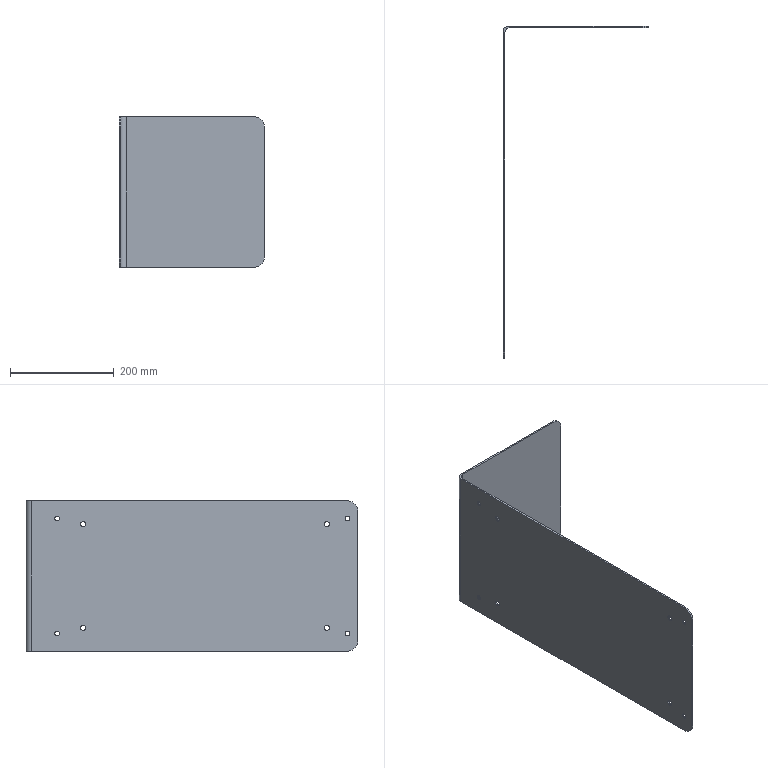Component | SolidWorks | 315InverterBracket()-1 | 1 solid | 30 faces | box 280 x 640 x 290 mm | volume 795054 mm3 | cylinder 22 | plane 8 | commonest cylinder face diameters 10 x8 9 x8 40 x4 20 x2 | material Plain Carbon Steel
STEP:
#1=COLOUR_RGB('',0.7922,0.8196,0.9333);
#2=FILL_AREA_STYLE_COLOUR('',#1);
#3=FILL_AREA_STYLE('',(#2));
#4=SURFACE_STYLE_FILL_AREA(#3);
#5=SURFACE_SIDE_STYLE('',(#4));
#6=SURFACE_STYLE_USAGE(.BOTH.,#5);
#7=PRESENTATION_STYLE_ASSIGNMENT((#6));
#8=CARTESIAN_POINT('',(26.575,78.937,-63.15));
#9=VERTEX_POINT('',#8);
#10=CARTESIAN_POINT('',(26.575,79.331,-63.15));
#11=VERTEX_POINT('',#10);
#12=CARTESIAN_POINT('',(26.575,79.134,-63.15));
#13=DIRECTION('',(-1.,0.,0.));
#14=DIRECTION('',(0.,-1.,0.));
#15=AXIS2_PLACEMENT_3D('',#12,#13,#14);
#16=CIRCLE('',#15,0.1969);
#17=EDGE_CURVE('',#9,#11,#16,.T.);
#18=ORIENTED_EDGE('',*,*,#17,.T.);
#19=CARTESIAN_POINT('',(26.693,79.331,-63.15));
#20=VERTEX_POINT('',#19);
#21=CARTESIAN_POINT('',(26.693,79.331,-63.15));
#22=DIRECTION('',(1.,-0.,-0.));
#23=VECTOR('',#22,39.37);
#24=LINE('',#21,#23);
#25=EDGE_CURVE('',#11,#20,#24,.T.);
#26=ORIENTED_EDGE('',*,*,#25,.T.);
#27=CARTESIAN_POINT('',(26.693,78.937,-63.15));
#28=VERTEX_POINT('',#27);
#29=CARTESIAN_POINT('',(26.693,79.134,-63.15));
#30=DIRECTION('',(-1.,0.,0.));
#31=DIRECTION('',(0.,-1.,0.));
#32=AXIS2_PLACEMENT_3D('',#29,#30,#31);
#33=CIRCLE('',#32,0.1969);
#34=EDGE_CURVE('',#28,#20,#33,.T.);
#35=ORIENTED_EDGE('',*,*,#34,.F.);
#36=CARTESIAN_POINT('',(26.693,78.937,-63.15));
#37=DIRECTION('',(1.,-0.,-0.));
#38=VECTOR('',#37,39.37);
#39=LINE('',#36,#38);
#40=EDGE_CURVE('',#9,#28,#39,.T.);
#41=ORIENTED_EDGE('',*,*,#40,.F.);
#42=EDGE_LOOP('',(#18,#26,#35,#41));
#43=FACE_OUTER_BOUND('',#42,.T.);
#44=CARTESIAN_POINT('',(26.693,79.134,-63.15));
#45=DIRECTION('',(1.,-0.,-0.));
#46=DIRECTION('',(0.,-1.,0.));
#47=AXIS2_PLACEMENT_3D('',#44,#45,#46);
#48=CYLINDRICAL_SURFACE('',#47,0.1969);
#49=ADVANCED_FACE('',(#43),#48,.F.);
#50=CARTESIAN_POINT('',(26.575,78.937,-71.024));
#51=VERTEX_POINT('',#50);
#52=CARTESIAN_POINT('',(26.575,79.331,-71.024));
#53=VERTEX_POINT('',#52);
#54=CARTESIAN_POINT('',(26.575,79.134,-71.024));
#55=DIRECTION('',(-1.,0.,0.));
#56=DIRECTION('',(0.,-1.,0.));
#57=AXIS2_PLACEMENT_3D('',#54,#55,#56);
#58=CIRCLE('',#57,0.1969);
#59=EDGE_CURVE('',#51,#53,#58,.T.);
#60=ORIENTED_EDGE('',*,*,#59,.T.);
#61=CARTESIAN_POINT('',(26.693,79.331,-71.024));
#62=VERTEX_POINT('',#61);
#63=CARTESIAN_POINT('',(26.693,79.331,-71.024));
#64=DIRECTION('',(1.,-0.,-0.));
#65=VECTOR('',#64,39.37);
#66=LINE('',#63,#65);
#67=EDGE_CURVE('',#53,#62,#66,.T.);
#68=ORIENTED_EDGE('',*,*,#67,.T.);
#69=CARTESIAN_POINT('',(26.693,78.937,-71.024));
#70=VERTEX_POINT('',#69);
#71=CARTESIAN_POINT('',(26.693,79.134,-71.024));
#72=DIRECTION('',(-1.,0.,0.));
#73=DIRECTION('',(0.,-1.,0.));
#74=AXIS2_PLACEMENT_3D('',#71,#72,#73);
#75=CIRCLE('',#74,0.1969);
#76=EDGE_CURVE('',#70,#62,#75,.T.);
#77=ORIENTED_EDGE('',*,*,#76,.F.);
#78=CARTESIAN_POINT('',(26.693,78.937,-71.024));
#79=DIRECTION('',(1.,-0.,-0.));
#80=VECTOR('',#79,39.37);
#81=LINE('',#78,#80);
#82=EDGE_CURVE('',#51,#70,#81,.T.);
#83=ORIENTED_EDGE('',*,*,#82,.F.);
#84=EDGE_LOOP('',(#60,#68,#77,#83));
#85=FACE_OUTER_BOUND('',#84,.T.);
#86=CARTESIAN_POINT('',(26.693,79.134,-71.024));
#87=DIRECTION('',(1.,-0.,-0.));
#88=DIRECTION('',(0.,-1.,0.));
#89=AXIS2_PLACEMENT_3D('',#86,#87,#88);
#90=CYLINDRICAL_SURFACE('',#89,0.1969);
#91=ADVANCED_FACE('',(#85),#90,.F.);
#92=CARTESIAN_POINT('',(26.575,97.441,-71.024));
#93=VERTEX_POINT('',#92);
#94=CARTESIAN_POINT('',(26.575,97.835,-71.024));
#95=VERTEX_POINT('',#94);
#96=CARTESIAN_POINT('',(26.575,97.638,-71.024));
#97=DIRECTION('',(-1.,0.,0.));
#98=DIRECTION('',(0.,-1.,0.));
#99=AXIS2_PLACEMENT_3D('',#96,#97,#98);
#100=CIRCLE('',#99,0.1969);
#101=EDGE_CURVE('',#93,#95,#100,.T.);
#102=ORIENTED_EDGE('',*,*,#101,.T.);
#103=CARTESIAN_POINT('',(26.693,97.835,-71.024));
#104=VERTEX_POINT('',#103);
#105=CARTESIAN_POINT('',(26.693,97.835,-71.024));
#106=DIRECTION('',(1.,-0.,-0.));
#107=VECTOR('',#106,39.37);
#108=LINE('',#105,#107);
#109=EDGE_CURVE('',#95,#104,#108,.T.);
#110=ORIENTED_EDGE('',*,*,#109,.T.);
#111=CARTESIAN_POINT('',(26.693,97.441,-71.024));
#112=VERTEX_POINT('',#111);
#113=CARTESIAN_POINT('',(26.693,97.638,-71.024));
#114=DIRECTION('',(-1.,0.,0.));
#115=DIRECTION('',(0.,-1.,0.));
#116=AXIS2_PLACEMENT_3D('',#113,#114,#115);
#117=CIRCLE('',#116,0.1969);
#118=EDGE_CURVE('',#112,#104,#117,.T.);
#119=ORIENTED_EDGE('',*,*,#118,.F.);
#120=CARTESIAN_POINT('',(26.693,97.441,-71.024));
#121=DIRECTION('',(1.,-0.,-0.));
#122=VECTOR('',#121,39.37);
#123=LINE('',#120,#122);
#124=EDGE_CURVE('',#93,#112,#123,.T.);
#125=ORIENTED_EDGE('',*,*,#124,.F.);
#126=EDGE_LOOP('',(#102,#110,#119,#125));
#127=FACE_OUTER_BOUND('',#126,.T.);
#128=CARTESIAN_POINT('',(26.693,97.638,-71.024));
#129=DIRECTION('',(1.,-0.,-0.));
#130=DIRECTION('',(0.,-1.,0.));
#131=AXIS2_PLACEMENT_3D('',#128,#129,#130);
#132=CYLINDRICAL_SURFACE('',#131,0.1969);
#133=ADVANCED_FACE('',(#127),#132,.F.);
#134=CARTESIAN_POINT('',(26.575,97.441,-63.15));
#135=VERTEX_POINT('',#134);
#136=CARTESIAN_POINT('',(26.575,97.835,-63.15));
#137=VERTEX_POINT('',#136);
#138=CARTESIAN_POINT('',(26.575,97.638,-63.15));
#139=DIRECTION('',(-1.,0.,0.));
#140=DIRECTION('',(0.,-1.,0.));
#141=AXIS2_PLACEMENT_3D('',#138,#139,#140);
#142=CIRCLE('',#141,0.1969);
#143=EDGE_CURVE('',#135,#137,#142,.T.);
#144=ORIENTED_EDGE('',*,*,#143,.T.);
#145=CARTESIAN_POINT('',(26.693,97.835,-63.15));
#146=VERTEX_POINT('',#145);
#147=CARTESIAN_POINT('',(26.693,97.835,-63.15));
#148=DIRECTION('',(1.,-0.,-0.));
#149=VECTOR('',#148,39.37);
#150=LINE('',#147,#149);
#151=EDGE_CURVE('',#137,#146,#150,.T.);
#152=ORIENTED_EDGE('',*,*,#151,.T.);
#153=CARTESIAN_POINT('',(26.693,97.441,-63.15));
#154=VERTEX_POINT('',#153);
#155=CARTESIAN_POINT('',(26.693,97.638,-63.15));
#156=DIRECTION('',(-1.,0.,0.));
#157=DIRECTION('',(0.,-1.,0.));
#158=AXIS2_PLACEMENT_3D('',#155,#156,#157);
#159=CIRCLE('',#158,0.1969);
#160=EDGE_CURVE('',#154,#146,#159,.T.);
#161=ORIENTED_EDGE('',*,*,#160,.F.);
#162=CARTESIAN_POINT('',(26.693,97.441,-63.15));
#163=DIRECTION('',(1.,-0.,-0.));
#164=VECTOR('',#163,39.37);
#165=LINE('',#162,#164);
#166=EDGE_CURVE('',#135,#154,#165,.T.);
#167=ORIENTED_EDGE('',*,*,#166,.F.);
#168=EDGE_LOOP('',(#144,#152,#161,#167));
#169=FACE_OUTER_BOUND('',#168,.T.);
#170=CARTESIAN_POINT('',(26.693,97.638,-63.15));
#171=DIRECTION('',(1.,-0.,-0.));
#172=DIRECTION('',(0.,-1.,0.));
#173=AXIS2_PLACEMENT_3D('',#170,#171,#172);
#174=CYLINDRICAL_SURFACE('',#173,0.1969);
#175=ADVANCED_FACE('',(#169),#174,.F.);
#176=CARTESIAN_POINT('',(26.575,77.382,-71.457));
#177=VERTEX_POINT('',#176);
#178=CARTESIAN_POINT('',(26.575,77.736,-71.457));
#179=VERTEX_POINT('',#178);
#180=CARTESIAN_POINT('',(26.575,77.559,-71.457));
#181=DIRECTION('',(-1.,0.,0.));
#182=DIRECTION('',(0.,-1.,0.));
#183=AXIS2_PLACEMENT_3D('',#180,#181,#182);
#184=CIRCLE('',#183,0.1772);
#185=EDGE_CURVE('',#177,#179,#184,.T.);
#186=ORIENTED_EDGE('',*,*,#185,.T.);
#187=CARTESIAN_POINT('',(26.693,77.736,-71.457));
#188=VERTEX_POINT('',#187);
#189=CARTESIAN_POINT('',(26.693,77.736,-71.457));
#190=DIRECTION('',(1.,-0.,-0.));
#191=VECTOR('',#190,39.37);
#192=LINE('',#189,#191);
#193=EDGE_CURVE('',#179,#188,#192,.T.);
#194=ORIENTED_EDGE('',*,*,#193,.T.);
#195=CARTESIAN_POINT('',(26.693,77.382,-71.457));
#196=VERTEX_POINT('',#195);
#197=CARTESIAN_POINT('',(26.693,77.559,-71.457));
#198=DIRECTION('',(-1.,0.,0.));
#199=DIRECTION('',(0.,-1.,0.));
#200=AXIS2_PLACEMENT_3D('',#197,#198,#199);
#201=CIRCLE('',#200,0.1772);
#202=EDGE_CURVE('',#196,#188,#201,.T.);
#203=ORIENTED_EDGE('',*,*,#202,.F.);
#204=CARTESIAN_POINT('',(26.693,77.382,-71.457));
#205=DIRECTION('',(1.,-0.,-0.));
#206=VECTOR('',#205,39.37);
#207=LINE('',#204,#206);
#208=EDGE_CURVE('',#177,#196,#207,.T.);
#209=ORIENTED_EDGE('',*,*,#208,.F.);
#210=EDGE_LOOP('',(#186,#194,#203,#209));
#211=FACE_OUTER_BOUND('',#210,.T.);
#212=CARTESIAN_POINT('',(26.693,77.559,-71.457));
#213=DIRECTION('',(1.,-0.,-0.));
#214=DIRECTION('',(0.,-1.,0.));
#215=AXIS2_PLACEMENT_3D('',#212,#213,#214);
#216=CYLINDRICAL_SURFACE('',#215,0.1772);
#217=ADVANCED_FACE('',(#211),#216,.F.);
#218=CARTESIAN_POINT('',(26.575,77.382,-62.717));
#219=VERTEX_POINT('',#218);
#220=CARTESIAN_POINT('',(26.575,77.736,-62.717));
#221=VERTEX_POINT('',#220);
#222=CARTESIAN_POINT('',(26.575,77.559,-62.717));
#223=DIRECTION('',(-1.,0.,0.));
#224=DIRECTION('',(0.,-1.,0.));
#225=AXIS2_PLACEMENT_3D('',#222,#223,#224);
#226=CIRCLE('',#225,0.1772);
#227=EDGE_CURVE('',#219,#221,#226,.T.);
#228=ORIENTED_EDGE('',*,*,#227,.T.);
#229=CARTESIAN_POINT('',(26.693,77.736,-62.717));
#230=VERTEX_POINT('',#229);
#231=CARTESIAN_POINT('',(26.693,77.736,-62.717));
#232=DIRECTION('',(1.,-0.,-0.));
#233=VECTOR('',#232,39.37);
#234=LINE('',#231,#233);
#235=EDGE_CURVE('',#221,#230,#234,.T.);
#236=ORIENTED_EDGE('',*,*,#235,.T.);
#237=CARTESIAN_POINT('',(26.693,77.382,-62.717));
#238=VERTEX_POINT('',#237);
#239=CARTESIAN_POINT('',(26.693,77.559,-62.717));
#240=DIRECTION('',(-1.,0.,0.));
#241=DIRECTION('',(0.,-1.,0.));
#242=AXIS2_PLACEMENT_3D('',#239,#240,#241);
#243=CIRCLE('',#242,0.1772);
#244=EDGE_CURVE('',#238,#230,#243,.T.);
#245=ORIENTED_EDGE('',*,*,#244,.F.);
#246=CARTESIAN_POINT('',(26.693,77.382,-62.717));
#247=DIRECTION('',(1.,-0.,-0.));
#248=VECTOR('',#247,39.37);
#249=LINE('',#246,#248);
#250=EDGE_CURVE('',#219,#238,#249,.T.);
#251=ORIENTED_EDGE('',*,*,#250,.F.);
#252=EDGE_LOOP('',(#228,#236,#245,#251));
#253=FACE_OUTER_BOUND('',#252,.T.);
#254=CARTESIAN_POINT('',(26.693,77.559,-62.717));
#255=DIRECTION('',(1.,-0.,-0.));
#256=DIRECTION('',(0.,-1.,0.));
#257=AXIS2_PLACEMENT_3D('',#254,#255,#256);
#258=CYLINDRICAL_SURFACE('',#257,0.1772);
#259=ADVANCED_FACE('',(#253),#258,.F.);
#260=CARTESIAN_POINT('',(26.575,99.429,-62.717));
#261=VERTEX_POINT('',#260);
#262=CARTESIAN_POINT('',(26.575,99.783,-62.717));
#263=VERTEX_POINT('',#262);
#264=CARTESIAN_POINT('',(26.575,99.606,-62.717));
#265=DIRECTION('',(-1.,0.,0.));
#266=DIRECTION('',(0.,-1.,0.));
#267=AXIS2_PLACEMENT_3D('',#264,#265,#266);
#268=CIRCLE('',#267,0.1772);
#269=EDGE_CURVE('',#261,#263,#268,.T.);
#270=ORIENTED_EDGE('',*,*,#269,.T.);
#271=CARTESIAN_POINT('',(26.693,99.783,-62.717));
#272=VERTEX_POINT('',#271);
#273=CARTESIAN_POINT('',(26.693,99.783,-62.717));
#274=DIRECTION('',(1.,-0.,-0.));
#275=VECTOR('',#274,39.37);
#276=LINE('',#273,#275);
#277=EDGE_CURVE('',#263,#272,#276,.T.);
#278=ORIENTED_EDGE('',*,*,#277,.T.);
#279=CARTESIAN_POINT('',(26.693,99.429,-62.717));
#280=VERTEX_POINT('',#279);
#281=CARTESIAN_POINT('',(26.693,99.606,-62.717));
#282=DIRECTION('',(-1.,0.,0.));
#283=DIRECTION('',(0.,-1.,0.));
#284=AXIS2_PLACEMENT_3D('',#281,#282,#283);
#285=CIRCLE('',#284,0.1772);
#286=EDGE_CURVE('',#280,#272,#285,.T.);
#287=ORIENTED_EDGE('',*,*,#286,.F.);
#288=CARTESIAN_POINT('',(26.693,99.429,-62.717));
#289=DIRECTION('',(1.,-0.,-0.));
#290=VECTOR('',#289,39.37);
#291=LINE('',#288,#290);
#292=EDGE_CURVE('',#261,#280,#291,.T.);
#293=ORIENTED_EDGE('',*,*,#292,.F.);
#294=EDGE_LOOP('',(#270,#278,#287,#293));
#295=FACE_OUTER_BOUND('',#294,.T.);
#296=CARTESIAN_POINT('',(26.693,99.606,-62.717));
#297=DIRECTION('',(1.,-0.,-0.));
#298=DIRECTION('',(0.,-1.,0.));
#299=AXIS2_PLACEMENT_3D('',#296,#297,#298);
#300=CYLINDRICAL_SURFACE('',#299,0.1772);
#301=ADVANCED_FACE('',(#295),#300,.F.);
#302=CARTESIAN_POINT('',(26.575,99.429,-71.457));
#303=VERTEX_POINT('',#302);
#304=CARTESIAN_POINT('',(26.575,99.783,-71.457));
#305=VERTEX_POINT('',#304);
#306=CARTESIAN_POINT('',(26.575,99.606,-71.457));
#307=DIRECTION('',(-1.,0.,0.));
#308=DIRECTION('',(0.,-1.,0.));
#309=AXIS2_PLACEMENT_3D('',#306,#307,#308);
#310=CIRCLE('',#309,0.1772);
#311=EDGE_CURVE('',#303,#305,#310,.T.);
#312=ORIENTED_EDGE('',*,*,#311,.T.);
#313=CARTESIAN_POINT('',(26.693,99.783,-71.457));
#314=VERTEX_POINT('',#313);
#315=CARTESIAN_POINT('',(26.693,99.783,-71.457));
#316=DIRECTION('',(1.,-0.,-0.));
#317=VECTOR('',#316,39.37);
#318=LINE('',#315,#317);
#319=EDGE_CURVE('',#305,#314,#318,.T.);
#320=ORIENTED_EDGE('',*,*,#319,.T.);
#321=CARTESIAN_POINT('',(26.693,99.429,-71.457));
#322=VERTEX_POINT('',#321);
#323=CARTESIAN_POINT('',(26.693,99.606,-71.457));
#324=DIRECTION('',(-1.,0.,0.));
#325=DIRECTION('',(0.,-1.,0.));
#326=AXIS2_PLACEMENT_3D('',#323,#324,#325);
#327=CIRCLE('',#326,0.1772);
#328=EDGE_CURVE('',#322,#314,#327,.T.);
#329=ORIENTED_EDGE('',*,*,#328,.F.);
#330=CARTESIAN_POINT('',(26.693,99.429,-71.457));
#331=DIRECTION('',(1.,-0.,-0.));
#332=VECTOR('',#331,39.37);
#333=LINE('',#330,#332);
#334=EDGE_CURVE('',#303,#322,#333,.T.);
#335=ORIENTED_EDGE('',*,*,#334,.F.);
#336=EDGE_LOOP('',(#312,#320,#329,#335));
#337=FACE_OUTER_BOUND('',#336,.T.);
#338=CARTESIAN_POINT('',(26.693,99.606,-71.457));
#339=DIRECTION('',(1.,-0.,-0.));
#340=DIRECTION('',(0.,-1.,0.));
#341=AXIS2_PLACEMENT_3D('',#338,#339,#340);
#342=CYLINDRICAL_SURFACE('',#341,0.1772);
#343=ADVANCED_FACE('',(#337),#342,.F.);
#344=CARTESIAN_POINT('',(26.575,76.772,-72.008));
#345=VERTEX_POINT('',#344);
#346=CARTESIAN_POINT('',(26.575,77.559,-72.795));
#347=VERTEX_POINT('',#346);
#348=CARTESIAN_POINT('',(26.575,77.559,-72.008));
#349=DIRECTION('',(1.,-0.,-0.));
#350=DIRECTION('',(0.,-1.,0.));
#351=AXIS2_PLACEMENT_3D('',#348,#349,#350);
#352=CIRCLE('',#351,0.7874);
#353=EDGE_CURVE('',#345,#347,#352,.T.);
#354=ORIENTED_EDGE('',*,*,#353,.F.);
#355=CARTESIAN_POINT('',(26.575,76.772,-62.165));
#356=VERTEX_POINT('',#355);
#357=CARTESIAN_POINT('',(26.575,76.772,-72.795));
#358=DIRECTION('',(-0.,0.,-1.));
#359=VECTOR('',#358,39.37);
#360=LINE('',#357,#359);
#361=EDGE_CURVE('',#356,#345,#360,.T.);
#362=ORIENTED_EDGE('',*,*,#361,.F.);
#363=CARTESIAN_POINT('',(26.575,77.559,-61.378));
#364=VERTEX_POINT('',#363);
#365=CARTESIAN_POINT('',(26.575,77.559,-62.165));
#366=DIRECTION('',(1.,-0.,-0.));
#367=DIRECTION('',(0.,1.,0.));
#368=AXIS2_PLACEMENT_3D('',#365,#366,#367);
#369=CIRCLE('',#368,0.7874);
#370=EDGE_CURVE('',#364,#356,#369,.T.);
#371=ORIENTED_EDGE('',*,*,#370,.F.);
#372=CARTESIAN_POINT('',(26.575,101.575,-61.378));
#373=VERTEX_POINT('',#372);
#374=CARTESIAN_POINT('',(26.575,76.772,-61.378));
#375=DIRECTION('',(-0.,-1.,-0.));
#376=VECTOR('',#375,39.37);
#377=LINE('',#374,#376);
#378=EDGE_CURVE('',#373,#364,#377,.T.);
#379=ORIENTED_EDGE('',*,*,#378,.F.);
#380=CARTESIAN_POINT('',(26.575,101.575,-72.795));
#381=VERTEX_POINT('',#380);
#382=CARTESIAN_POINT('',(26.575,101.575,-72.795));
#383=DIRECTION('',(0.,-0.,1.));
#384=VECTOR('',#383,39.37);
#385=LINE('',#382,#384);
#386=EDGE_CURVE('',#381,#373,#385,.T.);
#387=ORIENTED_EDGE('',*,*,#386,.F.);
#388=CARTESIAN_POINT('',(26.575,76.772,-72.795));
#389=DIRECTION('',(0.,1.,0.));
#390=VECTOR('',#389,39.37);
#391=LINE('',#388,#390);
#392=EDGE_CURVE('',#347,#381,#391,.T.);
#393=ORIENTED_EDGE('',*,*,#392,.F.);
#394=EDGE_LOOP('',(#354,#362,#371,#379,#387,#393));
#395=FACE_OUTER_BOUND('',#394,.T.);
#396=ORIENTED_EDGE('',*,*,#17,.F.);
#397=CARTESIAN_POINT('',(26.575,79.134,-63.15));
#398=DIRECTION('',(-1.,0.,0.));
#399=DIRECTION('',(0.,-1.,0.));
#400=AXIS2_PLACEMENT_3D('',#397,#398,#399);
#401=CIRCLE('',#400,0.1969);
#402=EDGE_CURVE('',#11,#9,#401,.T.);
#403=ORIENTED_EDGE('',*,*,#402,.F.);
#404=EDGE_LOOP('',(#396,#403));
#405=FACE_BOUND('',#404,.T.);
#406=ORIENTED_EDGE('',*,*,#59,.F.);
#407=CARTESIAN_POINT('',(26.575,79.134,-71.024));
#408=DIRECTION('',(-1.,0.,0.));
#409=DIRECTION('',(0.,-1.,0.));
#410=AXIS2_PLACEMENT_3D('',#407,#408,#409);
#411=CIRCLE('',#410,0.1969);
#412=EDGE_CURVE('',#53,#51,#411,.T.);
#413=ORIENTED_EDGE('',*,*,#412,.F.);
#414=EDGE_LOOP('',(#406,#413));
#415=FACE_BOUND('',#414,.T.);
#416=ORIENTED_EDGE('',*,*,#101,.F.);
#417=CARTESIAN_POINT('',(26.575,97.638,-71.024));
#418=DIRECTION('',(-1.,0.,0.));
#419=DIRECTION('',(0.,-1.,0.));
#420=AXIS2_PLACEMENT_3D('',#417,#418,#419);
#421=CIRCLE('',#420,0.1969);
#422=EDGE_CURVE('',#95,#93,#421,.T.);
#423=ORIENTED_EDGE('',*,*,#422,.F.);
#424=EDGE_LOOP('',(#416,#423));
#425=FACE_BOUND('',#424,.T.);
#426=ORIENTED_EDGE('',*,*,#143,.F.);
#427=CARTESIAN_POINT('',(26.575,97.638,-63.15));
#428=DIRECTION('',(-1.,0.,0.));
#429=DIRECTION('',(0.,-1.,0.));
#430=AXIS2_PLACEMENT_3D('',#427,#428,#429);
#431=CIRCLE('',#430,0.1969);
#432=EDGE_CURVE('',#137,#135,#431,.T.);
#433=ORIENTED_EDGE('',*,*,#432,.F.);
#434=EDGE_LOOP('',(#426,#433));
#435=FACE_BOUND('',#434,.T.);
#436=ORIENTED_EDGE('',*,*,#185,.F.);
#437=CARTESIAN_POINT('',(26.575,77.559,-71.457));
#438=DIRECTION('',(-1.,0.,0.));
#439=DIRECTION('',(0.,-1.,0.));
#440=AXIS2_PLACEMENT_3D('',#437,#438,#439);
#441=CIRCLE('',#440,0.1772);
#442=EDGE_CURVE('',#179,#177,#441,.T.);
#443=ORIENTED_EDGE('',*,*,#442,.F.);
#444=EDGE_LOOP('',(#436,#443));
#445=FACE_BOUND('',#444,.T.);
#446=ORIENTED_EDGE('',*,*,#227,.F.);
#447=CARTESIAN_POINT('',(26.575,77.559,-62.717));
#448=DIRECTION('',(-1.,0.,0.));
#449=DIRECTION('',(0.,-1.,0.));
#450=AXIS2_PLACEMENT_3D('',#447,#448,#449);
#451=CIRCLE('',#450,0.1772);
#452=EDGE_CURVE('',#221,#219,#451,.T.);
#453=ORIENTED_EDGE('',*,*,#452,.F.);
#454=EDGE_LOOP('',(#446,#453));
#455=FACE_BOUND('',#454,.T.);
#456=ORIENTED_EDGE('',*,*,#269,.F.);
#457=CARTESIAN_POINT('',(26.575,99.606,-62.717));
#458=DIRECTION('',(-1.,0.,0.));
#459=DIRECTION('',(0.,-1.,0.));
#460=AXIS2_PLACEMENT_3D('',#457,#458,#459);
#461=CIRCLE('',#460,0.1772);
#462=EDGE_CURVE('',#263,#261,#461,.T.);
#463=ORIENTED_EDGE('',*,*,#462,.F.);
#464=EDGE_LOOP('',(#456,#463));
#465=FACE_BOUND('',#464,.T.);
#466=ORIENTED_EDGE('',*,*,#311,.F.);
#467=CARTESIAN_POINT('',(26.575,99.606,-71.457));
#468=DIRECTION('',(-1.,0.,0.));
#469=DIRECTION('',(0.,-1.,0.));
#470=AXIS2_PLACEMENT_3D('',#467,#468,#469);
#471=CIRCLE('',#470,0.1772);
#472=EDGE_CURVE('',#305,#303,#471,.T.);
#473=ORIENTED_EDGE('',*,*,#472,.F.);
#474=EDGE_LOOP('',(#466,#473));
#475=FACE_BOUND('',#474,.T.);
#476=CARTESIAN_POINT('',(26.575,76.772,-72.795));
#477=DIRECTION('',(1.,-0.,-0.));
#478=DIRECTION('',(-0.,-1.,-0.));
#479=AXIS2_PLACEMENT_3D('',#476,#477,#478);
#480=PLANE('',#479);
#481=ADVANCED_FACE('',(#395,#405,#415,#425,#435,#445,#455,#465,#475),#480,.F.);
#482=CARTESIAN_POINT('',(36.811,101.85,-72.795));
#483=VERTEX_POINT('',#482);
#484=CARTESIAN_POINT('',(27.087,101.85,-72.795));
#485=VERTEX_POINT('',#484);
#486=CARTESIAN_POINT('',(26.969,101.85,-72.795));
#487=DIRECTION('',(-1.,0.,0.));
#488=VECTOR('',#487,39.37);
#489=LINE('',#486,#488);
#490=EDGE_CURVE('',#483,#485,#489,.T.);
#491=ORIENTED_EDGE('',*,*,#490,.T.);
#492=CARTESIAN_POINT('',(26.693,101.457,-72.795));
#493=VERTEX_POINT('',#492);
#494=CARTESIAN_POINT('',(27.087,101.457,-72.795));
#495=DIRECTION('',(0.,-0.,1.));
#496=DIRECTION('',(0.,1.,0.));
#497=AXIS2_PLACEMENT_3D('',#494,#495,#496);
#498=CIRCLE('',#497,0.3937);
#499=EDGE_CURVE('',#485,#493,#498,.T.);
#500=ORIENTED_EDGE('',*,*,#499,.T.);
#501=CARTESIAN_POINT('',(26.693,77.559,-72.795));
#502=VERTEX_POINT('',#501);
#503=CARTESIAN_POINT('',(26.693,101.575,-72.795));
#504=DIRECTION('',(-0.,-1.,-0.));
#505=VECTOR('',#504,39.37);
#506=LINE('',#503,#505);
#507=EDGE_CURVE('',#493,#502,#506,.T.);
#508=ORIENTED_EDGE('',*,*,#507,.T.);
#509=CARTESIAN_POINT('',(26.969,77.559,-72.795));
#510=DIRECTION('',(-1.,0.,0.));
#511=VECTOR('',#510,39.37);
#512=LINE('',#509,#511);
#513=EDGE_CURVE('',#502,#347,#512,.T.);
#514=ORIENTED_EDGE('',*,*,#513,.T.);
#515=ORIENTED_EDGE('',*,*,#392,.T.);
#516=CARTESIAN_POINT('',(26.969,101.969,-72.795));
#517=VERTEX_POINT('',#516);
#518=CARTESIAN_POINT('',(26.969,101.575,-72.795));
#519=DIRECTION('',(-0.,0.,-1.));
#520=DIRECTION('',(0.,1.,0.));
#521=AXIS2_PLACEMENT_3D('',#518,#519,#520);
#522=CIRCLE('',#521,0.3937);
#523=EDGE_CURVE('',#381,#517,#522,.T.);
#524=ORIENTED_EDGE('',*,*,#523,.T.);
#525=CARTESIAN_POINT('',(36.811,101.969,-72.795));
#526=VERTEX_POINT('',#525);
#527=CARTESIAN_POINT('',(26.969,101.969,-72.795));
#528=DIRECTION('',(1.,-0.,-0.));
#529=VECTOR('',#528,39.37);
#530=LINE('',#527,#529);
#531=EDGE_CURVE('',#517,#526,#530,.T.);
#532=ORIENTED_EDGE('',*,*,#531,.T.);
#533=CARTESIAN_POINT('',(36.811,101.575,-72.795));
#534=DIRECTION('',(-0.,-1.,-0.));
#535=VECTOR('',#534,39.37);
#536=LINE('',#533,#535);
#537=EDGE_CURVE('',#526,#483,#536,.T.);
#538=ORIENTED_EDGE('',*,*,#537,.T.);
#539=EDGE_LOOP('',(#491,#500,#508,#514,#515,#524,#532,#538));
#540=FACE_OUTER_BOUND('',#539,.T.);
#541=CARTESIAN_POINT('',(26.969,101.575,-72.795));
#542=DIRECTION('',(-0.,0.,-1.));
#543=DIRECTION('',(-0.,-1.,-0.));
#544=AXIS2_PLACEMENT_3D('',#541,#542,#543);
#545=PLANE('',#544);
#546=ADVANCED_FACE('',(#540),#545,.T.);
#547=ORIENTED_EDGE('',*,*,#353,.T.);
#548=ORIENTED_EDGE('',*,*,#513,.F.);
#549=CARTESIAN_POINT('',(26.693,76.772,-72.008));
#550=VERTEX_POINT('',#549);
#551=CARTESIAN_POINT('',(26.693,77.559,-72.008));
#552=DIRECTION('',(-1.,0.,0.));
#553=DIRECTION('',(0.,-1.,0.));
#554=AXIS2_PLACEMENT_3D('',#551,#552,#553);
#555=CIRCLE('',#554,0.7874);
#556=EDGE_CURVE('',#502,#550,#555,.T.);
#557=ORIENTED_EDGE('',*,*,#556,.T.);
#558=CARTESIAN_POINT('',(26.969,76.772,-72.008));
#559=DIRECTION('',(-1.,0.,0.));
#560=VECTOR('',#559,39.37);
#561=LINE('',#558,#560);
#562=EDGE_CURVE('',#550,#345,#561,.T.);
#563=ORIENTED_EDGE('',*,*,#562,.T.);
#564=EDGE_LOOP('',(#547,#548,#557,#563));
#565=FACE_OUTER_BOUND('',#564,.T.);
#566=CARTESIAN_POINT('',(26.969,77.559,-72.008));
#567=DIRECTION('',(1.,-0.,-0.));
#568=DIRECTION('',(0.,-1.,0.));
#569=AXIS2_PLACEMENT_3D('',#566,#567,#568);
#570=CYLINDRICAL_SURFACE('',#569,0.7874);
#571=ADVANCED_FACE('',(#565),#570,.T.);
#572=ORIENTED_EDGE('',*,*,#562,.F.);
#573=CARTESIAN_POINT('',(26.693,76.772,-62.165));
#574=VERTEX_POINT('',#573);
#575=CARTESIAN_POINT('',(26.693,76.772,-72.795));
#576=DIRECTION('',(-0.,0.,-1.));
#577=VECTOR('',#576,39.37);
#578=LINE('',#575,#577);
#579=EDGE_CURVE('',#574,#550,#578,.T.);
#580=ORIENTED_EDGE('',*,*,#579,.F.);
#581=CARTESIAN_POINT('',(26.693,76.772,-62.165));
#582=DIRECTION('',(1.,-0.,-0.));
#583=VECTOR('',#582,39.37);
#584=LINE('',#581,#583);
#585=EDGE_CURVE('',#356,#574,#584,.T.);
#586=ORIENTED_EDGE('',*,*,#585,.F.);
#587=ORIENTED_EDGE('',*,*,#361,.T.);
#588=EDGE_LOOP('',(#572,#580,#586,#587));
#589=FACE_OUTER_BOUND('',#588,.T.);
#590=CARTESIAN_POINT('',(26.693,76.772,-72.795));
#591=DIRECTION('',(0.,1.,0.));
#592=DIRECTION('',(1.,-0.,-0.));
#593=AXIS2_PLACEMENT_3D('',#590,#591,#592);
#594=PLANE('',#593);
#595=ADVANCED_FACE('',(#589),#594,.F.);
#596=ORIENTED_EDGE('',*,*,#370,.T.);
#597=ORIENTED_EDGE('',*,*,#585,.T.);
#598=CARTESIAN_POINT('',(26.693,77.559,-61.378));
#599=VERTEX_POINT('',#598);
#600=CARTESIAN_POINT('',(26.693,77.559,-62.165));
#601=DIRECTION('',(-1.,0.,0.));
#602=DIRECTION('',(0.,1.,0.));
#603=AXIS2_PLACEMENT_3D('',#600,#601,#602);
#604=CIRCLE('',#603,0.7874);
#605=EDGE_CURVE('',#574,#599,#604,.T.);
#606=ORIENTED_EDGE('',*,*,#605,.T.);
#607=CARTESIAN_POINT('',(26.693,77.559,-61.378));
#608=DIRECTION('',(-1.,0.,0.));
#609=VECTOR('',#608,39.37);
#610=LINE('',#607,#609);
#611=EDGE_CURVE('',#599,#364,#610,.T.);
#612=ORIENTED_EDGE('',*,*,#611,.T.);
#613=EDGE_LOOP('',(#596,#597,#606,#612));
#614=FACE_OUTER_BOUND('',#613,.T.);
#615=CARTESIAN_POINT('',(26.693,77.559,-62.165));
#616=DIRECTION('',(-1.,0.,0.));
#617=DIRECTION('',(0.,1.,0.));
#618=AXIS2_PLACEMENT_3D('',#615,#616,#617);
#619=CYLINDRICAL_SURFACE('',#618,0.7874);
#620=ADVANCED_FACE('',(#614),#619,.T.);
#621=ORIENTED_EDGE('',*,*,#611,.F.);
#622=CARTESIAN_POINT('',(26.693,101.457,-61.378));
#623=VERTEX_POINT('',#622);
#624=CARTESIAN_POINT('',(26.693,101.575,-61.378));
#625=DIRECTION('',(-0.,-1.,-0.));
#626=VECTOR('',#625,39.37);
#627=LINE('',#624,#626);
#628=EDGE_CURVE('',#623,#599,#627,.T.);
#629=ORIENTED_EDGE('',*,*,#628,.F.);
#630=CARTESIAN_POINT('',(27.087,101.85,-61.378));
#631=VERTEX_POINT('',#630);
#632=CARTESIAN_POINT('',(27.087,101.457,-61.378));
#633=DIRECTION('',(0.,-0.,1.));
#634=DIRECTION('',(0.,1.,0.));
#635=AXIS2_PLACEMENT_3D('',#632,#633,#634);
#636=CIRCLE('',#635,0.3937);
#637=EDGE_CURVE('',#631,#623,#636,.T.);
#638=ORIENTED_EDGE('',*,*,#637,.F.);
#639=CARTESIAN_POINT('',(36.811,101.85,-61.378));
#640=VERTEX_POINT('',#639);
#641=CARTESIAN_POINT('',(26.969,101.85,-61.378));
#642=DIRECTION('',(-1.,0.,0.));
#643=VECTOR('',#642,39.37);
#644=LINE('',#641,#643);
#645=EDGE_CURVE('',#640,#631,#644,.T.);
#646=ORIENTED_EDGE('',*,*,#645,.F.);
#647=CARTESIAN_POINT('',(36.811,101.969,-61.378));
#648=VERTEX_POINT('',#647);
#649=CARTESIAN_POINT('',(36.811,101.575,-61.378));
#650=DIRECTION('',(-0.,-1.,-0.));
#651=VECTOR('',#650,39.37);
#652=LINE('',#649,#651);
#653=EDGE_CURVE('',#648,#640,#652,.T.);
#654=ORIENTED_EDGE('',*,*,#653,.F.);
#655=CARTESIAN_POINT('',(26.969,101.969,-61.378));
#656=VERTEX_POINT('',#655);
#657=CARTESIAN_POINT('',(26.969,101.969,-61.378));
#658=DIRECTION('',(1.,-0.,-0.));
#659=VECTOR('',#658,39.37);
#660=LINE('',#657,#659);
#661=EDGE_CURVE('',#656,#648,#660,.T.);
#662=ORIENTED_EDGE('',*,*,#661,.F.);
#663=CARTESIAN_POINT('',(26.969,101.575,-61.378));
#664=DIRECTION('',(-0.,0.,-1.));
#665=DIRECTION('',(0.,1.,0.));
#666=AXIS2_PLACEMENT_3D('',#663,#664,#665);
#667=CIRCLE('',#666,0.3937);
#668=EDGE_CURVE('',#373,#656,#667,.T.);
#669=ORIENTED_EDGE('',*,*,#668,.F.);
#670=ORIENTED_EDGE('',*,*,#378,.T.);
#671=EDGE_LOOP('',(#621,#629,#638,#646,#654,#662,#669,#670));
#672=FACE_OUTER_BOUND('',#671,.T.);
#673=CARTESIAN_POINT('',(26.969,101.575,-61.378));
#674=DIRECTION('',(-0.,0.,-1.));
#675=DIRECTION('',(-0.,-1.,-0.));
#676=AXIS2_PLACEMENT_3D('',#673,#674,#675);
#677=PLANE('',#676);
#678=ADVANCED_FACE('',(#672),#677,.F.);
#679=ORIENTED_EDGE('',*,*,#523,.F.);
#680=ORIENTED_EDGE('',*,*,#386,.T.);
#681=ORIENTED_EDGE('',*,*,#668,.T.);
#682=CARTESIAN_POINT('',(26.969,101.969,-72.795));
#683=DIRECTION('',(-0.,0.,-1.));
#684=VECTOR('',#683,39.37);
#685=LINE('',#682,#684);
#686=EDGE_CURVE('',#656,#517,#685,.T.);
#687=ORIENTED_EDGE('',*,*,#686,.T.);
#688=EDGE_LOOP('',(#679,#680,#681,#687));
#689=FACE_OUTER_BOUND('',#688,.T.);
#690=CARTESIAN_POINT('',(26.969,101.575,-72.795));
#691=DIRECTION('',(0.,-0.,1.));
#692=DIRECTION('',(0.,1.,0.));
#693=AXIS2_PLACEMENT_3D('',#690,#691,#692);
#694=CYLINDRICAL_SURFACE('',#693,0.3937);
#695=ADVANCED_FACE('',(#689),#694,.T.);
#696=ORIENTED_EDGE('',*,*,#25,.F.);
#697=ORIENTED_EDGE('',*,*,#402,.T.);
#698=ORIENTED_EDGE('',*,*,#40,.T.);
#699=CARTESIAN_POINT('',(26.693,79.134,-63.15));
#700=DIRECTION('',(-1.,0.,0.));
#701=DIRECTION('',(0.,-1.,0.));
#702=AXIS2_PLACEMENT_3D('',#699,#700,#701);
#703=CIRCLE('',#702,0.1969);
#704=EDGE_CURVE('',#20,#28,#703,.T.);
#705=ORIENTED_EDGE('',*,*,#704,.F.);
#706=EDGE_LOOP('',(#696,#697,#698,#705));
#707=FACE_OUTER_BOUND('',#706,.T.);
#708=CARTESIAN_POINT('',(26.693,79.134,-63.15));
#709=DIRECTION('',(1.,-0.,-0.));
#710=DIRECTION('',(0.,-1.,0.));
#711=AXIS2_PLACEMENT_3D('',#708,#709,#710);
#712=CYLINDRICAL_SURFACE('',#711,0.1969);
#713=ADVANCED_FACE('',(#707),#712,.F.);
#714=ORIENTED_EDGE('',*,*,#67,.F.);
#715=ORIENTED_EDGE('',*,*,#412,.T.);
#716=ORIENTED_EDGE('',*,*,#82,.T.);
#717=CARTESIAN_POINT('',(26.693,79.134,-71.024));
#718=DIRECTION('',(-1.,0.,0.));
#719=DIRECTION('',(0.,-1.,0.));
#720=AXIS2_PLACEMENT_3D('',#717,#718,#719);
#721=CIRCLE('',#720,0.1969);
#722=EDGE_CURVE('',#62,#70,#721,.T.);
#723=ORIENTED_EDGE('',*,*,#722,.F.);
#724=EDGE_LOOP('',(#714,#715,#716,#723));
#725=FACE_OUTER_BOUND('',#724,.T.);
#726=CARTESIAN_POINT('',(26.693,79.134,-71.024));
#727=DIRECTION('',(1.,-0.,-0.));
#728=DIRECTION('',(0.,-1.,0.));
#729=AXIS2_PLACEMENT_3D('',#726,#727,#728);
#730=CYLINDRICAL_SURFACE('',#729,0.1969);
#731=ADVANCED_FACE('',(#725),#730,.F.);
#732=ORIENTED_EDGE('',*,*,#109,.F.);
#733=ORIENTED_EDGE('',*,*,#422,.T.);
#734=ORIENTED_EDGE('',*,*,#124,.T.);
#735=CARTESIAN_POINT('',(26.693,97.638,-71.024));
#736=DIRECTION('',(-1.,0.,0.));
#737=DIRECTION('',(0.,-1.,0.));
#738=AXIS2_PLACEMENT_3D('',#735,#736,#737);
#739=CIRCLE('',#738,0.1969);
#740=EDGE_CURVE('',#104,#112,#739,.T.);
#741=ORIENTED_EDGE('',*,*,#740,.F.);
#742=EDGE_LOOP('',(#732,#733,#734,#741));
#743=FACE_OUTER_BOUND('',#742,.T.);
#744=CARTESIAN_POINT('',(26.693,97.638,-71.024));
#745=DIRECTION('',(1.,-0.,-0.));
#746=DIRECTION('',(0.,-1.,0.));
#747=AXIS2_PLACEMENT_3D('',#744,#745,#746);
#748=CYLINDRICAL_SURFACE('',#747,0.1969);
#749=ADVANCED_FACE('',(#743),#748,.F.);
#750=ORIENTED_EDGE('',*,*,#151,.F.);
#751=ORIENTED_EDGE('',*,*,#432,.T.);
#752=ORIENTED_EDGE('',*,*,#166,.T.);
#753=CARTESIAN_POINT('',(26.693,97.638,-63.15));
#754=DIRECTION('',(-1.,0.,0.));
#755=DIRECTION('',(0.,-1.,0.));
#756=AXIS2_PLACEMENT_3D('',#753,#754,#755);
#757=CIRCLE('',#756,0.1969);
#758=EDGE_CURVE('',#146,#154,#757,.T.);
#759=ORIENTED_EDGE('',*,*,#758,.F.);
#760=EDGE_LOOP('',(#750,#751,#752,#759));
#761=FACE_OUTER_BOUND('',#760,.T.);
#762=CARTESIAN_POINT('',(26.693,97.638,-63.15));
#763=DIRECTION('',(1.,-0.,-0.));
#764=DIRECTION('',(0.,-1.,0.));
#765=AXIS2_PLACEMENT_3D('',#762,#763,#764);
#766=CYLINDRICAL_SURFACE('',#765,0.1969);
#767=ADVANCED_FACE('',(#761),#766,.F.);
#768=ORIENTED_EDGE('',*,*,#193,.F.);
#769=ORIENTED_EDGE('',*,*,#442,.T.);
#770=ORIENTED_EDGE('',*,*,#208,.T.);
#771=CARTESIAN_POINT('',(26.693,77.559,-71.457));
#772=DIRECTION('',(-1.,0.,0.));
#773=DIRECTION('',(0.,-1.,0.));
#774=AXIS2_PLACEMENT_3D('',#771,#772,#773);
#775=CIRCLE('',#774,0.1772);
#776=EDGE_CURVE('',#188,#196,#775,.T.);
#777=ORIENTED_EDGE('',*,*,#776,.F.);
#778=EDGE_LOOP('',(#768,#769,#770,#777));
#779=FACE_OUTER_BOUND('',#778,.T.);
#780=CARTESIAN_POINT('',(26.693,77.559,-71.457));
#781=DIRECTION('',(1.,-0.,-0.));
#782=DIRECTION('',(0.,-1.,0.));
#783=AXIS2_PLACEMENT_3D('',#780,#781,#782);
#784=CYLINDRICAL_SURFACE('',#783,0.1772);
#785=ADVANCED_FACE('',(#779),#784,.F.);
#786=ORIENTED_EDGE('',*,*,#235,.F.);
#787=ORIENTED_EDGE('',*,*,#452,.T.);
#788=ORIENTED_EDGE('',*,*,#250,.T.);
#789=CARTESIAN_POINT('',(26.693,77.559,-62.717));
#790=DIRECTION('',(-1.,0.,0.));
#791=DIRECTION('',(0.,-1.,0.));
#792=AXIS2_PLACEMENT_3D('',#789,#790,#791);
#793=CIRCLE('',#792,0.1772);
#794=EDGE_CURVE('',#230,#238,#793,.T.);
#795=ORIENTED_EDGE('',*,*,#794,.F.);
#796=EDGE_LOOP('',(#786,#787,#788,#795));
#797=FACE_OUTER_BOUND('',#796,.T.);
#798=CARTESIAN_POINT('',(26.693,77.559,-62.717));
#799=DIRECTION('',(1.,-0.,-0.));
#800=DIRECTION('',(0.,-1.,0.));
#801=AXIS2_PLACEMENT_3D('',#798,#799,#800);
#802=CYLINDRICAL_SURFACE('',#801,0.1772);
#803=ADVANCED_FACE('',(#797),#802,.F.);
#804=ORIENTED_EDGE('',*,*,#277,.F.);
#805=ORIENTED_EDGE('',*,*,#462,.T.);
#806=ORIENTED_EDGE('',*,*,#292,.T.);
#807=CARTESIAN_POINT('',(26.693,99.606,-62.717));
#808=DIRECTION('',(-1.,0.,0.));
#809=DIRECTION('',(0.,-1.,0.));
#810=AXIS2_PLACEMENT_3D('',#807,#808,#809);
#811=CIRCLE('',#810,0.1772);
#812=EDGE_CURVE('',#272,#280,#811,.T.);
#813=ORIENTED_EDGE('',*,*,#812,.F.);
#814=EDGE_LOOP('',(#804,#805,#806,#813));
#815=FACE_OUTER_BOUND('',#814,.T.);
#816=CARTESIAN_POINT('',(26.693,99.606,-62.717));
#817=DIRECTION('',(1.,-0.,-0.));
#818=DIRECTION('',(0.,-1.,0.));
#819=AXIS2_PLACEMENT_3D('',#816,#817,#818);
#820=CYLINDRICAL_SURFACE('',#819,0.1772);
#821=ADVANCED_FACE('',(#815),#820,.F.);
#822=ORIENTED_EDGE('',*,*,#319,.F.);
#823=ORIENTED_EDGE('',*,*,#472,.T.);
#824=ORIENTED_EDGE('',*,*,#334,.T.);
#825=CARTESIAN_POINT('',(26.693,99.606,-71.457));
#826=DIRECTION('',(-1.,0.,0.));
#827=DIRECTION('',(0.,-1.,0.));
#828=AXIS2_PLACEMENT_3D('',#825,#826,#827);
#829=CIRCLE('',#828,0.1772);
#830=EDGE_CURVE('',#314,#322,#829,.T.);
#831=ORIENTED_EDGE('',*,*,#830,.F.);
#832=EDGE_LOOP('',(#822,#823,#824,#831));
#833=FACE_OUTER_BOUND('',#832,.T.);
#834=CARTESIAN_POINT('',(26.693,99.606,-71.457));
#835=DIRECTION('',(1.,-0.,-0.));
#836=DIRECTION('',(0.,-1.,0.));
#837=AXIS2_PLACEMENT_3D('',#834,#835,#836);
#838=CYLINDRICAL_SURFACE('',#837,0.1772);
#839=ADVANCED_FACE('',(#833),#838,.F.);
#840=CARTESIAN_POINT('',(26.693,101.457,-72.795));
#841=DIRECTION('',(0.,-0.,1.));
#842=VECTOR('',#841,39.37);
#843=LINE('',#840,#842);
#844=EDGE_CURVE('',#493,#623,#843,.T.);
#845=ORIENTED_EDGE('',*,*,#844,.F.);
#846=ORIENTED_EDGE('',*,*,#499,.F.);
#847=CARTESIAN_POINT('',(27.087,101.85,-72.795));
#848=DIRECTION('',(-0.,0.,-1.));
#849=VECTOR('',#848,39.37);
#850=LINE('',#847,#849);
#851=EDGE_CURVE('',#631,#485,#850,.T.);
#852=ORIENTED_EDGE('',*,*,#851,.F.);
#853=ORIENTED_EDGE('',*,*,#637,.T.);
#854=EDGE_LOOP('',(#845,#846,#852,#853));
#855=FACE_OUTER_BOUND('',#854,.T.);
#856=CARTESIAN_POINT('',(27.087,101.457,-72.795));
#857=DIRECTION('',(0.,-0.,1.));
#858=DIRECTION('',(0.,1.,0.));
#859=AXIS2_PLACEMENT_3D('',#856,#857,#858);
#860=CYLINDRICAL_SURFACE('',#859,0.3937);
#861=ADVANCED_FACE('',(#855),#860,.F.);
#862=CARTESIAN_POINT('',(37.598,101.85,-62.165));
#863=VERTEX_POINT('',#862);
#864=CARTESIAN_POINT('',(36.811,101.85,-62.165));
#865=DIRECTION('',(0.,1.,0.));
#866=DIRECTION('',(-1.,0.,0.));
#867=AXIS2_PLACEMENT_3D('',#864,#865,#866);
#868=CIRCLE('',#867,0.7874);
#869=EDGE_CURVE('',#640,#863,#868,.T.);
#870=ORIENTED_EDGE('',*,*,#869,.F.);
#871=ORIENTED_EDGE('',*,*,#645,.T.);
#872=ORIENTED_EDGE('',*,*,#851,.T.);
#873=ORIENTED_EDGE('',*,*,#490,.F.);
#874=CARTESIAN_POINT('',(37.598,101.85,-72.008));
#875=VERTEX_POINT('',#874);
#876=CARTESIAN_POINT('',(36.811,101.85,-72.008));
#877=DIRECTION('',(0.,1.,0.));
#878=DIRECTION('',(1.,0.,0.));
#879=AXIS2_PLACEMENT_3D('',#876,#877,#878);
#880=CIRCLE('',#879,0.7874);
#881=EDGE_CURVE('',#875,#483,#880,.T.);
#882=ORIENTED_EDGE('',*,*,#881,.F.);
#883=CARTESIAN_POINT('',(37.598,101.85,-72.795));
#884=DIRECTION('',(-0.,0.,-1.));
#885=VECTOR('',#884,39.37);
#886=LINE('',#883,#885);
#887=EDGE_CURVE('',#863,#875,#886,.T.);
#888=ORIENTED_EDGE('',*,*,#887,.F.);
#889=EDGE_LOOP('',(#870,#871,#872,#873,#882,#888));
#890=FACE_OUTER_BOUND('',#889,.T.);
#891=CARTESIAN_POINT('',(37.598,101.85,-72.795));
#892=DIRECTION('',(0.,1.,0.));
#893=DIRECTION('',(1.,-0.,-0.));
#894=AXIS2_PLACEMENT_3D('',#891,#892,#893);
#895=PLANE('',#894);
#896=ADVANCED_FACE('',(#890),#895,.F.);
#897=ORIENTED_EDGE('',*,*,#881,.T.);
#898=ORIENTED_EDGE('',*,*,#537,.F.);
#899=CARTESIAN_POINT('',(37.598,101.969,-72.008));
#900=VERTEX_POINT('',#899);
#901=CARTESIAN_POINT('',(36.811,101.969,-72.008));
#902=DIRECTION('',(-0.,-1.,-0.));
#903=DIRECTION('',(1.,0.,0.));
#904=AXIS2_PLACEMENT_3D('',#901,#902,#903);
#905=CIRCLE('',#904,0.7874);
#906=EDGE_CURVE('',#526,#900,#905,.T.);
#907=ORIENTED_EDGE('',*,*,#906,.T.);
#908=CARTESIAN_POINT('',(37.598,101.575,-72.008));
#909=DIRECTION('',(-0.,-1.,-0.));
#910=VECTOR('',#909,39.37);
#911=LINE('',#908,#910);
#912=EDGE_CURVE('',#900,#875,#911,.T.);
#913=ORIENTED_EDGE('',*,*,#912,.T.);
#914=EDGE_LOOP('',(#897,#898,#907,#913));
#915=FACE_OUTER_BOUND('',#914,.T.);
#916=CARTESIAN_POINT('',(36.811,101.575,-72.008));
#917=DIRECTION('',(0.,1.,0.));
#918=DIRECTION('',(1.,0.,0.));
#919=AXIS2_PLACEMENT_3D('',#916,#917,#918);
#920=CYLINDRICAL_SURFACE('',#919,0.7874);
#921=ADVANCED_FACE('',(#915),#920,.T.);
#922=CARTESIAN_POINT('',(37.598,101.969,-62.165));
#923=VERTEX_POINT('',#922);
#924=CARTESIAN_POINT('',(36.811,101.969,-62.165));
#925=DIRECTION('',(-0.,-1.,-0.));
#926=DIRECTION('',(-1.,0.,0.));
#927=AXIS2_PLACEMENT_3D('',#924,#925,#926);
#928=CIRCLE('',#927,0.7874);
#929=EDGE_CURVE('',#923,#648,#928,.T.);
#930=ORIENTED_EDGE('',*,*,#929,.F.);
#931=CARTESIAN_POINT('',(37.598,101.969,-72.795));
#932=DIRECTION('',(0.,-0.,1.));
#933=VECTOR('',#932,39.37);
#934=LINE('',#931,#933);
#935=EDGE_CURVE('',#900,#923,#934,.T.);
#936=ORIENTED_EDGE('',*,*,#935,.F.);
#937=ORIENTED_EDGE('',*,*,#906,.F.);
#938=ORIENTED_EDGE('',*,*,#531,.F.);
#939=ORIENTED_EDGE('',*,*,#686,.F.);
#940=ORIENTED_EDGE('',*,*,#661,.T.);
#941=EDGE_LOOP('',(#930,#936,#937,#938,#939,#940));
#942=FACE_OUTER_BOUND('',#941,.T.);
#943=CARTESIAN_POINT('',(26.969,101.969,-72.795));
#944=DIRECTION('',(-0.,-1.,-0.));
#945=DIRECTION('',(-1.,0.,0.));
#946=AXIS2_PLACEMENT_3D('',#943,#944,#945);
#947=PLANE('',#946);
#948=ADVANCED_FACE('',(#942),#947,.F.);
#949=ORIENTED_EDGE('',*,*,#556,.F.);
#950=ORIENTED_EDGE('',*,*,#507,.F.);
#951=ORIENTED_EDGE('',*,*,#844,.T.);
#952=ORIENTED_EDGE('',*,*,#628,.T.);
#953=ORIENTED_EDGE('',*,*,#605,.F.);
#954=ORIENTED_EDGE('',*,*,#579,.T.);
#955=EDGE_LOOP('',(#949,#950,#951,#952,#953,#954));
#956=FACE_OUTER_BOUND('',#955,.T.);
#957=ORIENTED_EDGE('',*,*,#34,.T.);
#958=ORIENTED_EDGE('',*,*,#704,.T.);
#959=EDGE_LOOP('',(#957,#958));
#960=FACE_BOUND('',#959,.T.);
#961=ORIENTED_EDGE('',*,*,#76,.T.);
#962=ORIENTED_EDGE('',*,*,#722,.T.);
#963=EDGE_LOOP('',(#961,#962));
#964=FACE_BOUND('',#963,.T.);
#965=ORIENTED_EDGE('',*,*,#118,.T.);
#966=ORIENTED_EDGE('',*,*,#740,.T.);
#967=EDGE_LOOP('',(#965,#966));
#968=FACE_BOUND('',#967,.T.);
#969=ORIENTED_EDGE('',*,*,#160,.T.);
#970=ORIENTED_EDGE('',*,*,#758,.T.);
#971=EDGE_LOOP('',(#969,#970));
#972=FACE_BOUND('',#971,.T.);
#973=ORIENTED_EDGE('',*,*,#202,.T.);
#974=ORIENTED_EDGE('',*,*,#776,.T.);
#975=EDGE_LOOP('',(#973,#974));
#976=FACE_BOUND('',#975,.T.);
#977=ORIENTED_EDGE('',*,*,#244,.T.);
#978=ORIENTED_EDGE('',*,*,#794,.T.);
#979=EDGE_LOOP('',(#977,#978));
#980=FACE_BOUND('',#979,.T.);
#981=ORIENTED_EDGE('',*,*,#286,.T.);
#982=ORIENTED_EDGE('',*,*,#812,.T.);
#983=EDGE_LOOP('',(#981,#982));
#984=FACE_BOUND('',#983,.T.);
#985=ORIENTED_EDGE('',*,*,#328,.T.);
#986=ORIENTED_EDGE('',*,*,#830,.T.);
#987=EDGE_LOOP('',(#985,#986));
#988=FACE_BOUND('',#987,.T.);
#989=CARTESIAN_POINT('',(26.693,101.457,-72.795));
#990=DIRECTION('',(-1.,0.,0.));
#991=DIRECTION('',(0.,1.,0.));
#992=AXIS2_PLACEMENT_3D('',#989,#990,#991);
#993=PLANE('',#992);
#994=ADVANCED_FACE('',(#956,#960,#964,#968,#972,#976,#980,#984,#988),#993,.F.);
#995=ORIENTED_EDGE('',*,*,#869,.T.);
#996=CARTESIAN_POINT('',(37.598,101.969,-62.165));
#997=DIRECTION('',(0.,1.,0.));
#998=VECTOR('',#997,39.37);
#999=LINE('',#996,#998);
#1000=EDGE_CURVE('',#863,#923,#999,.T.);
#1001=ORIENTED_EDGE('',*,*,#1000,.T.);
#1002=ORIENTED_EDGE('',*,*,#929,.T.);
#1003=ORIENTED_EDGE('',*,*,#653,.T.);
#1004=EDGE_LOOP('',(#995,#1001,#1002,#1003));
#1005=FACE_OUTER_BOUND('',#1004,.T.);
#1006=CARTESIAN_POINT('',(36.811,101.969,-62.165));
#1007=DIRECTION('',(-0.,-1.,-0.));
#1008=DIRECTION('',(-1.,0.,0.));
#1009=AXIS2_PLACEMENT_3D('',#1006,#1007,#1008);
#1010=CYLINDRICAL_SURFACE('',#1009,0.7874);
#1011=ADVANCED_FACE('',(#1005),#1010,.T.);
#1012=ORIENTED_EDGE('',*,*,#1000,.F.);
#1013=ORIENTED_EDGE('',*,*,#887,.T.);
#1014=ORIENTED_EDGE('',*,*,#912,.F.);
#1015=ORIENTED_EDGE('',*,*,#935,.T.);
#1016=EDGE_LOOP('',(#1012,#1013,#1014,#1015));
#1017=FACE_OUTER_BOUND('',#1016,.T.);
#1018=CARTESIAN_POINT('',(37.598,101.969,-72.795));
#1019=DIRECTION('',(-1.,0.,0.));
#1020=DIRECTION('',(0.,1.,0.));
#1021=AXIS2_PLACEMENT_3D('',#1018,#1019,#1020);
#1022=PLANE('',#1021);
#1023=ADVANCED_FACE('',(#1017),#1022,.F.);
#1024=CLOSED_SHELL('',(#49,#91,#133,#175,#217,#259,#301,#343,#481,#546,#571,#595,#620,#678,#695,#713,#731,#749,#767,#785,#803,#821,#839,#861,#896,#921,#948,#994,#1011,#1023));
#1025=MANIFOLD_SOLID_BREP('',#1024);
#1026=STYLED_ITEM('',(#7),#1025);
#1027=(LENGTH_UNIT()NAMED_UNIT(*)SI_UNIT($,.METRE.));
#1028=LENGTH_MEASURE_WITH_UNIT(LENGTH_MEASURE(0.0254),#1027);
#1029=DIMENSIONAL_EXPONENTS(1.,0.,0.,0.,0.,0.,0.);
#1030=(CONVERSION_BASED_UNIT('',#1028)LENGTH_UNIT()NAMED_UNIT(#1029));
#1031=UNCERTAINTY_MEASURE_WITH_UNIT(LENGTH_MEASURE(0.00001),#1030,'','');
#1032=(NAMED_UNIT(*)PLANE_ANGLE_UNIT()SI_UNIT($,.RADIAN.));
#1033=(NAMED_UNIT(*)SI_UNIT($,.STERADIAN.)SOLID_ANGLE_UNIT());
#1034=(GEOMETRIC_REPRESENTATION_CONTEXT(3)GLOBAL_UNCERTAINTY_ASSIGNED_CONTEXT((#1031))GLOBAL_UNIT_ASSIGNED_CONTEXT((#1030,#1032,#1033))REPRESENTATION_CONTEXT('',''));
#1035=MECHANICAL_DESIGN_GEOMETRIC_PRESENTATION_REPRESENTATION('',(#1026),#1034);
#1036=PRESENTATION_LAYER_ASSIGNMENT('','',(#1026));
#1037=CARTESIAN_POINT('',(0.,0.,0.));
#1038=DIRECTION('',(0.,0.,1.));
#1039=DIRECTION('',(1.,0.,0.));
#1040=AXIS2_PLACEMENT_3D('',#1037,#1038,#1039);
#1041=(LENGTH_UNIT()NAMED_UNIT(*)SI_UNIT($,.METRE.));
#1042=LENGTH_MEASURE_WITH_UNIT(LENGTH_MEASURE(0.0254),#1041);
#1043=DIMENSIONAL_EXPONENTS(1.,0.,0.,0.,0.,0.,0.);
#1044=(CONVERSION_BASED_UNIT('',#1042)LENGTH_UNIT()NAMED_UNIT(#1043));
#1045=UNCERTAINTY_MEASURE_WITH_UNIT(LENGTH_MEASURE(0.00001),#1044,'','');
#1046=(NAMED_UNIT(*)PLANE_ANGLE_UNIT()SI_UNIT($,.RADIAN.));
#1047=(NAMED_UNIT(*)SI_UNIT($,.STERADIAN.)SOLID_ANGLE_UNIT());
#1048=(GEOMETRIC_REPRESENTATION_CONTEXT(3)GLOBAL_UNCERTAINTY_ASSIGNED_CONTEXT((#1045))GLOBAL_UNIT_ASSIGNED_CONTEXT((#1044,#1046,#1047))REPRESENTATION_CONTEXT('',''));
#1049=ADVANCED_BREP_SHAPE_REPRESENTATION('',(#1025,#1040),#1048);